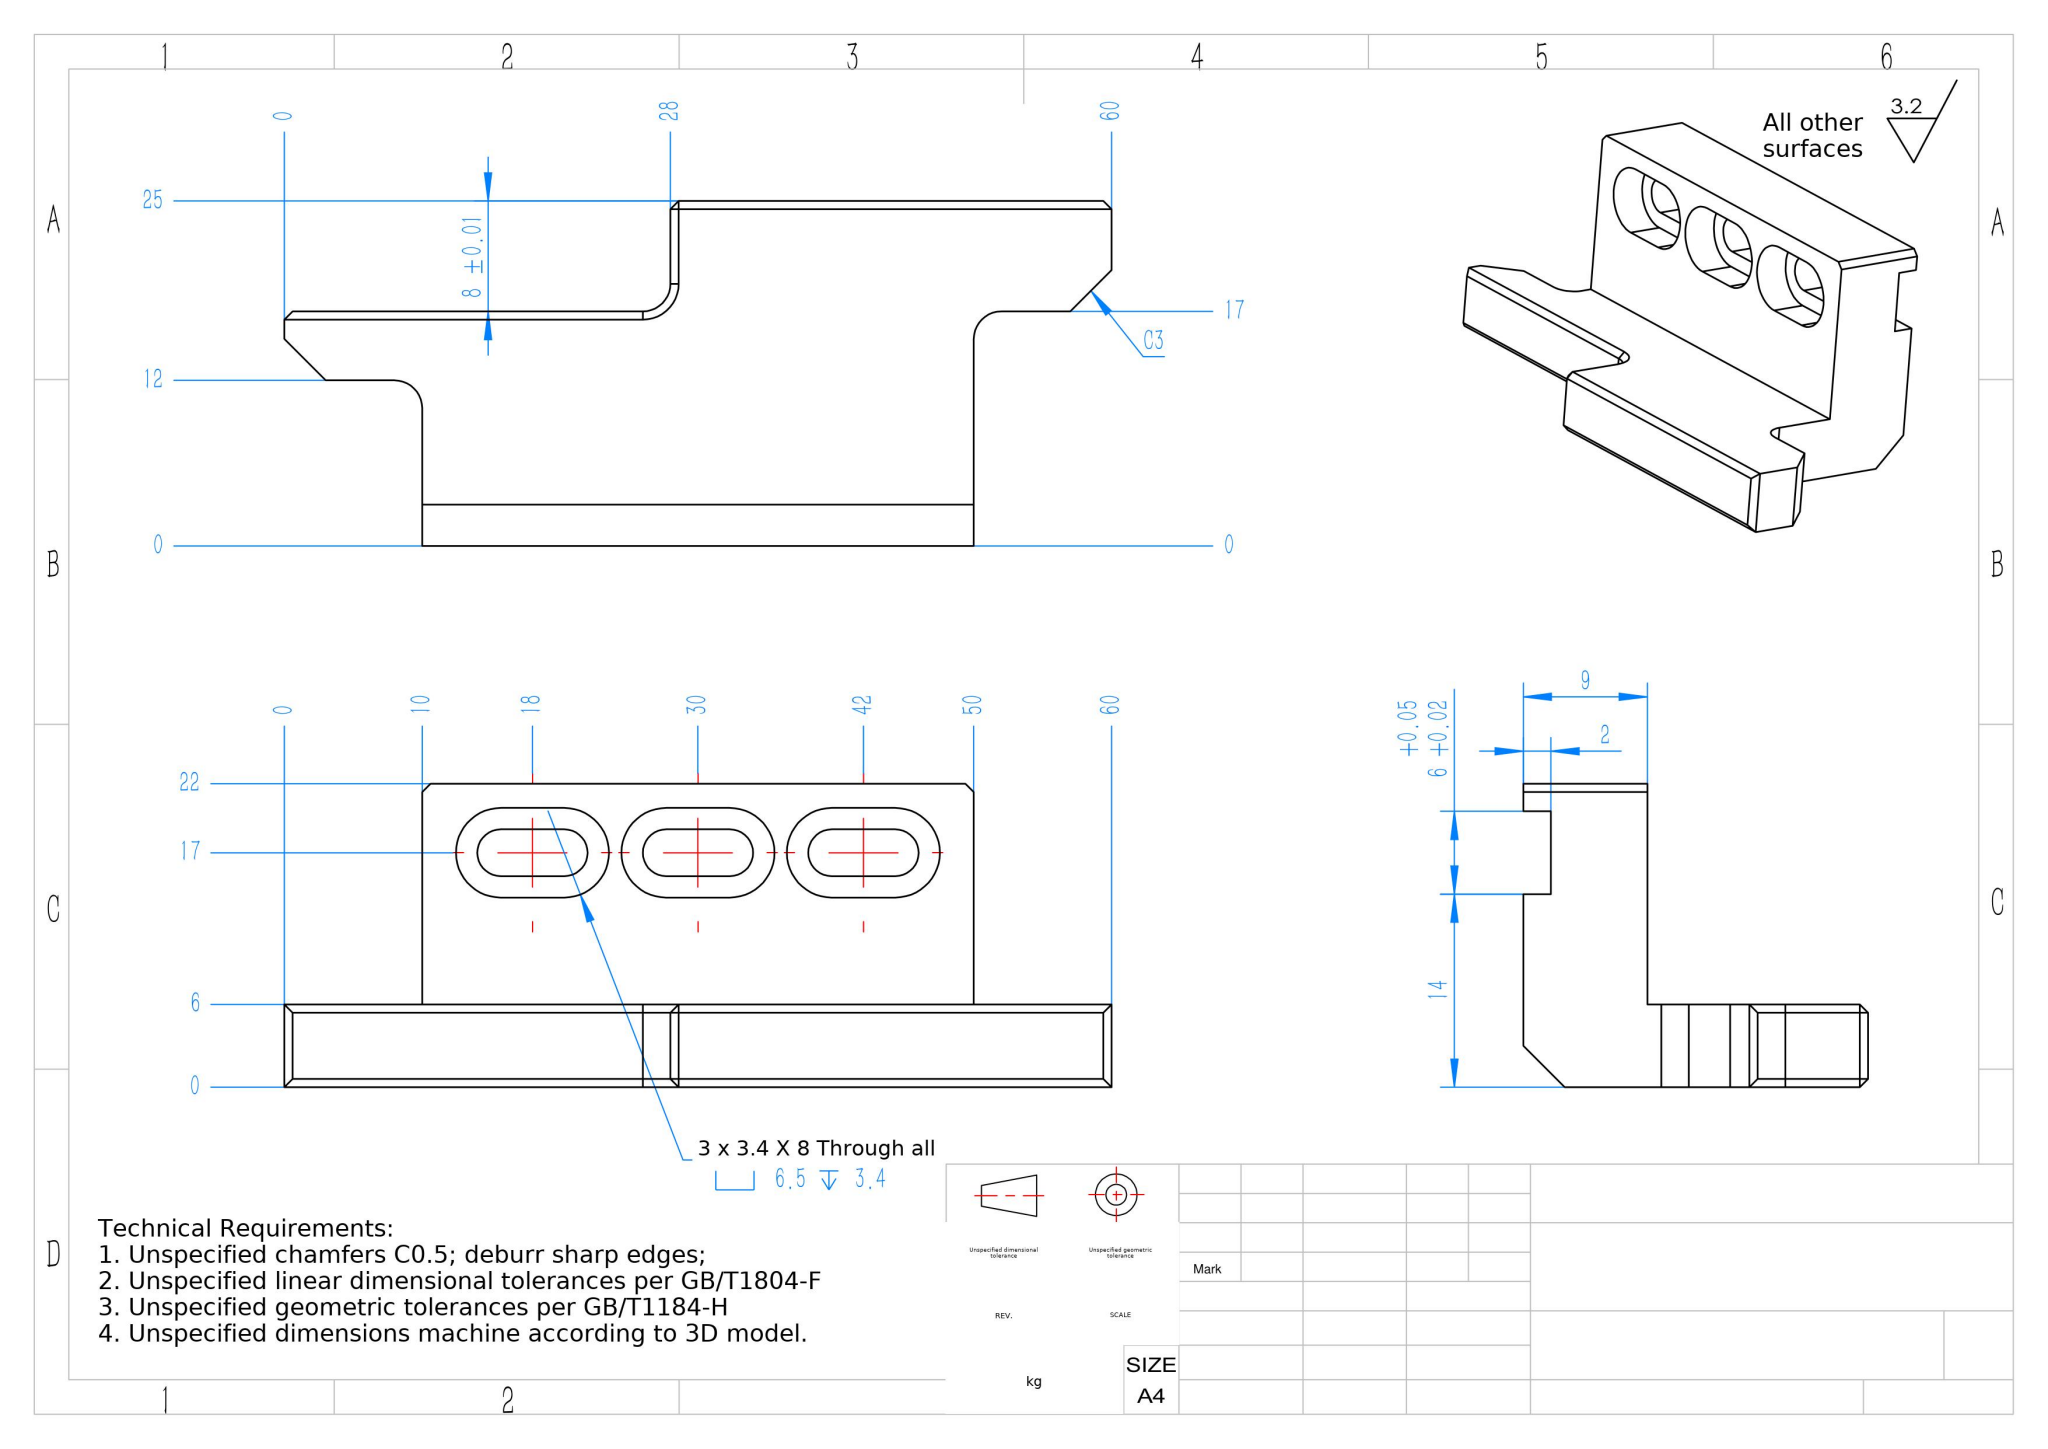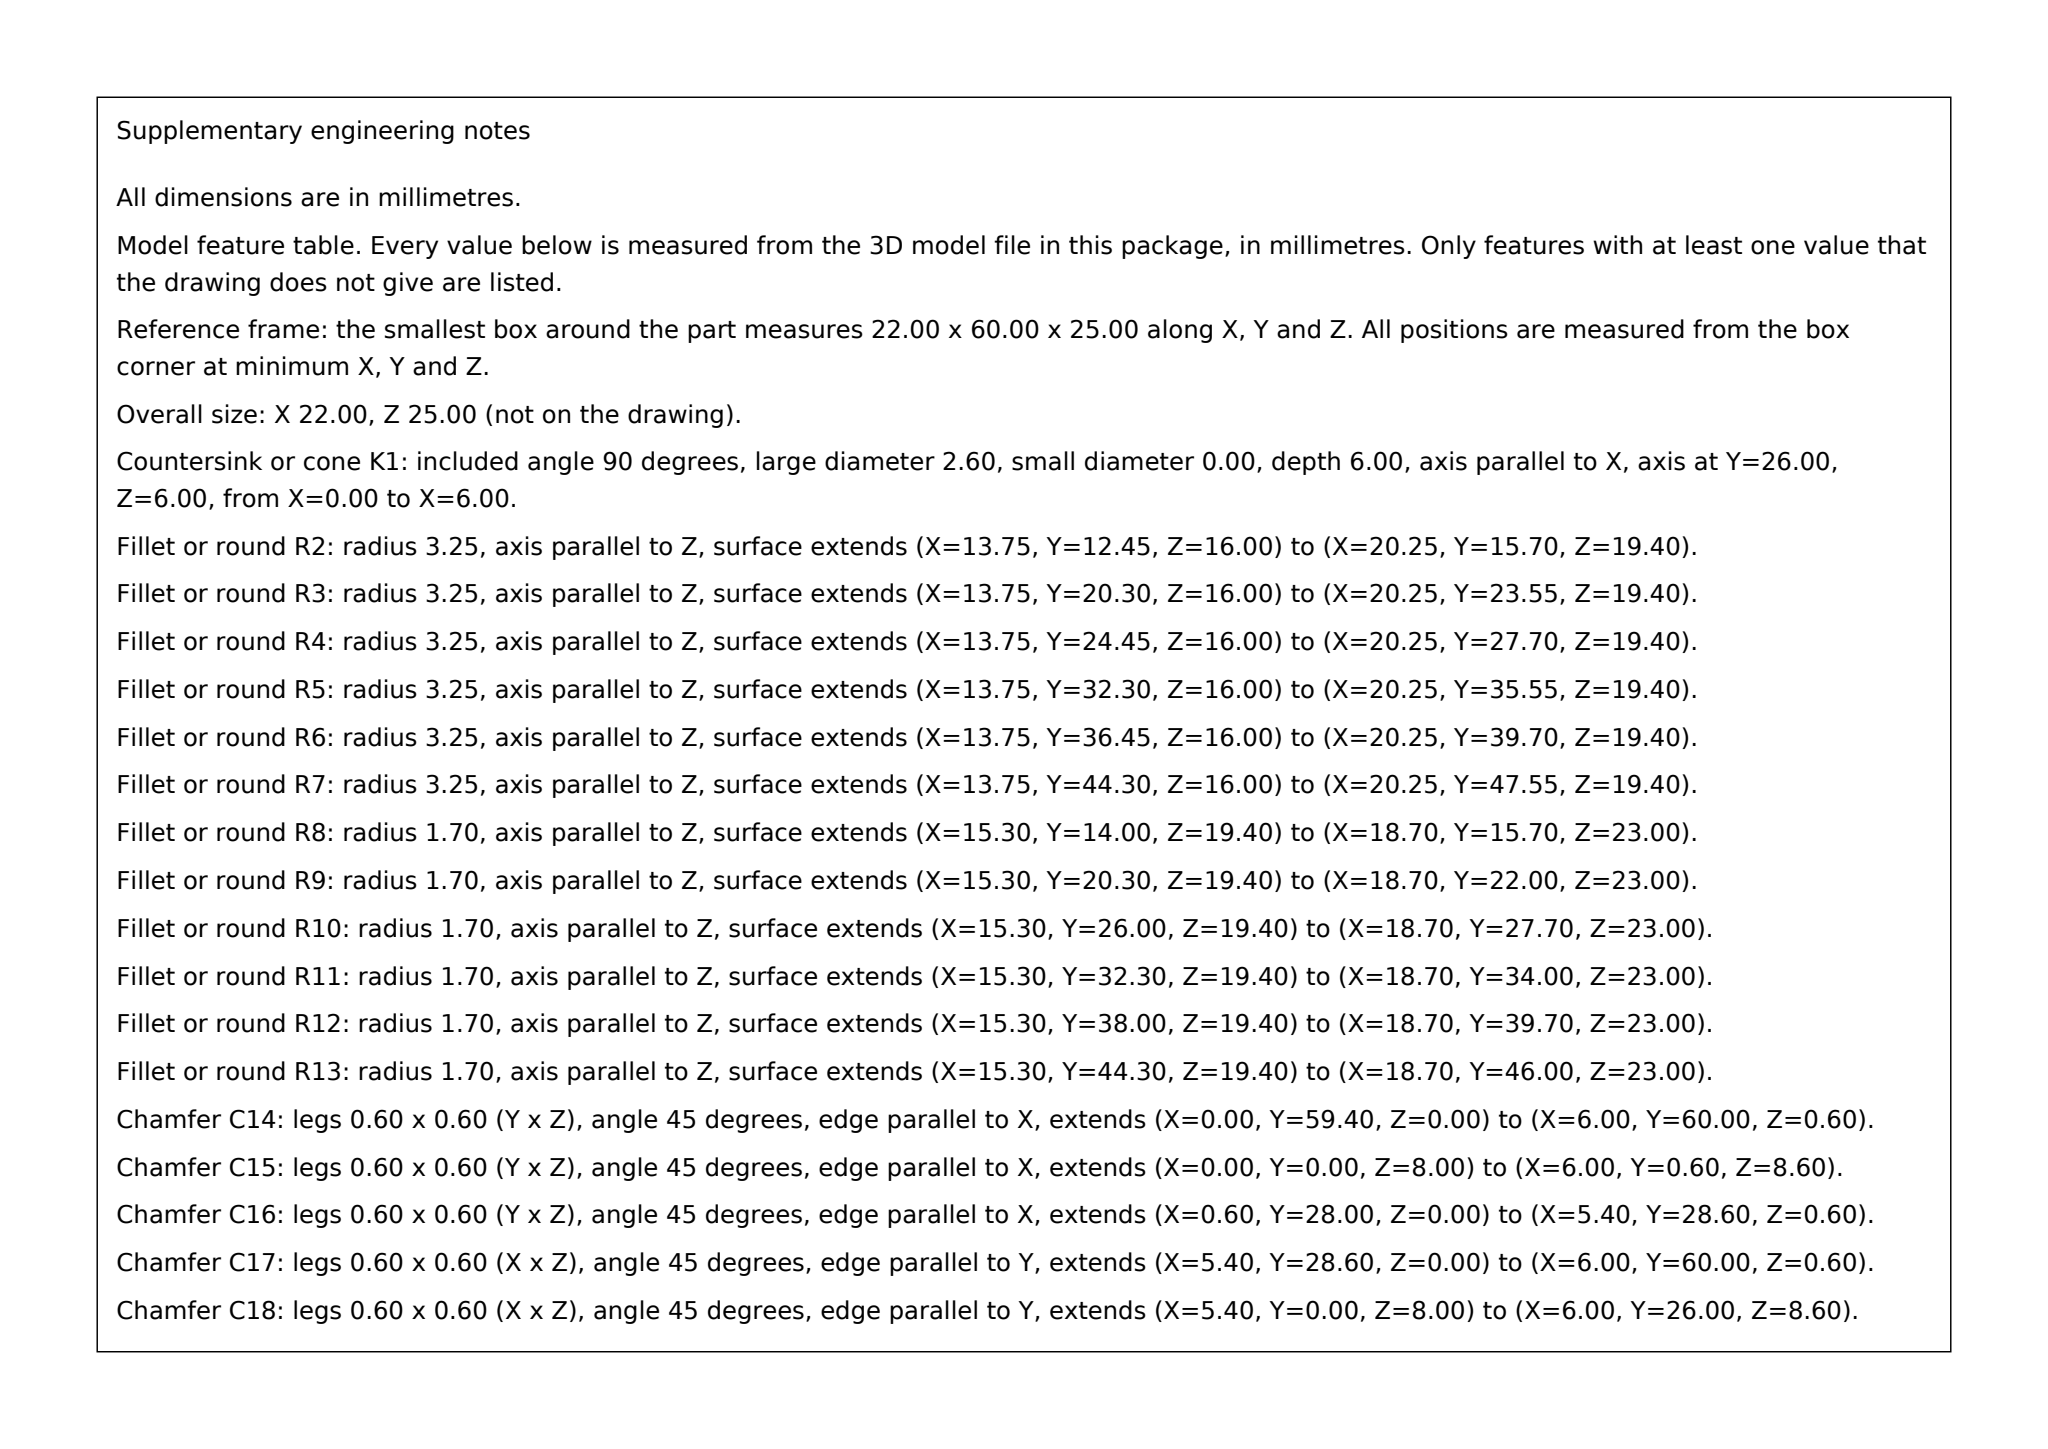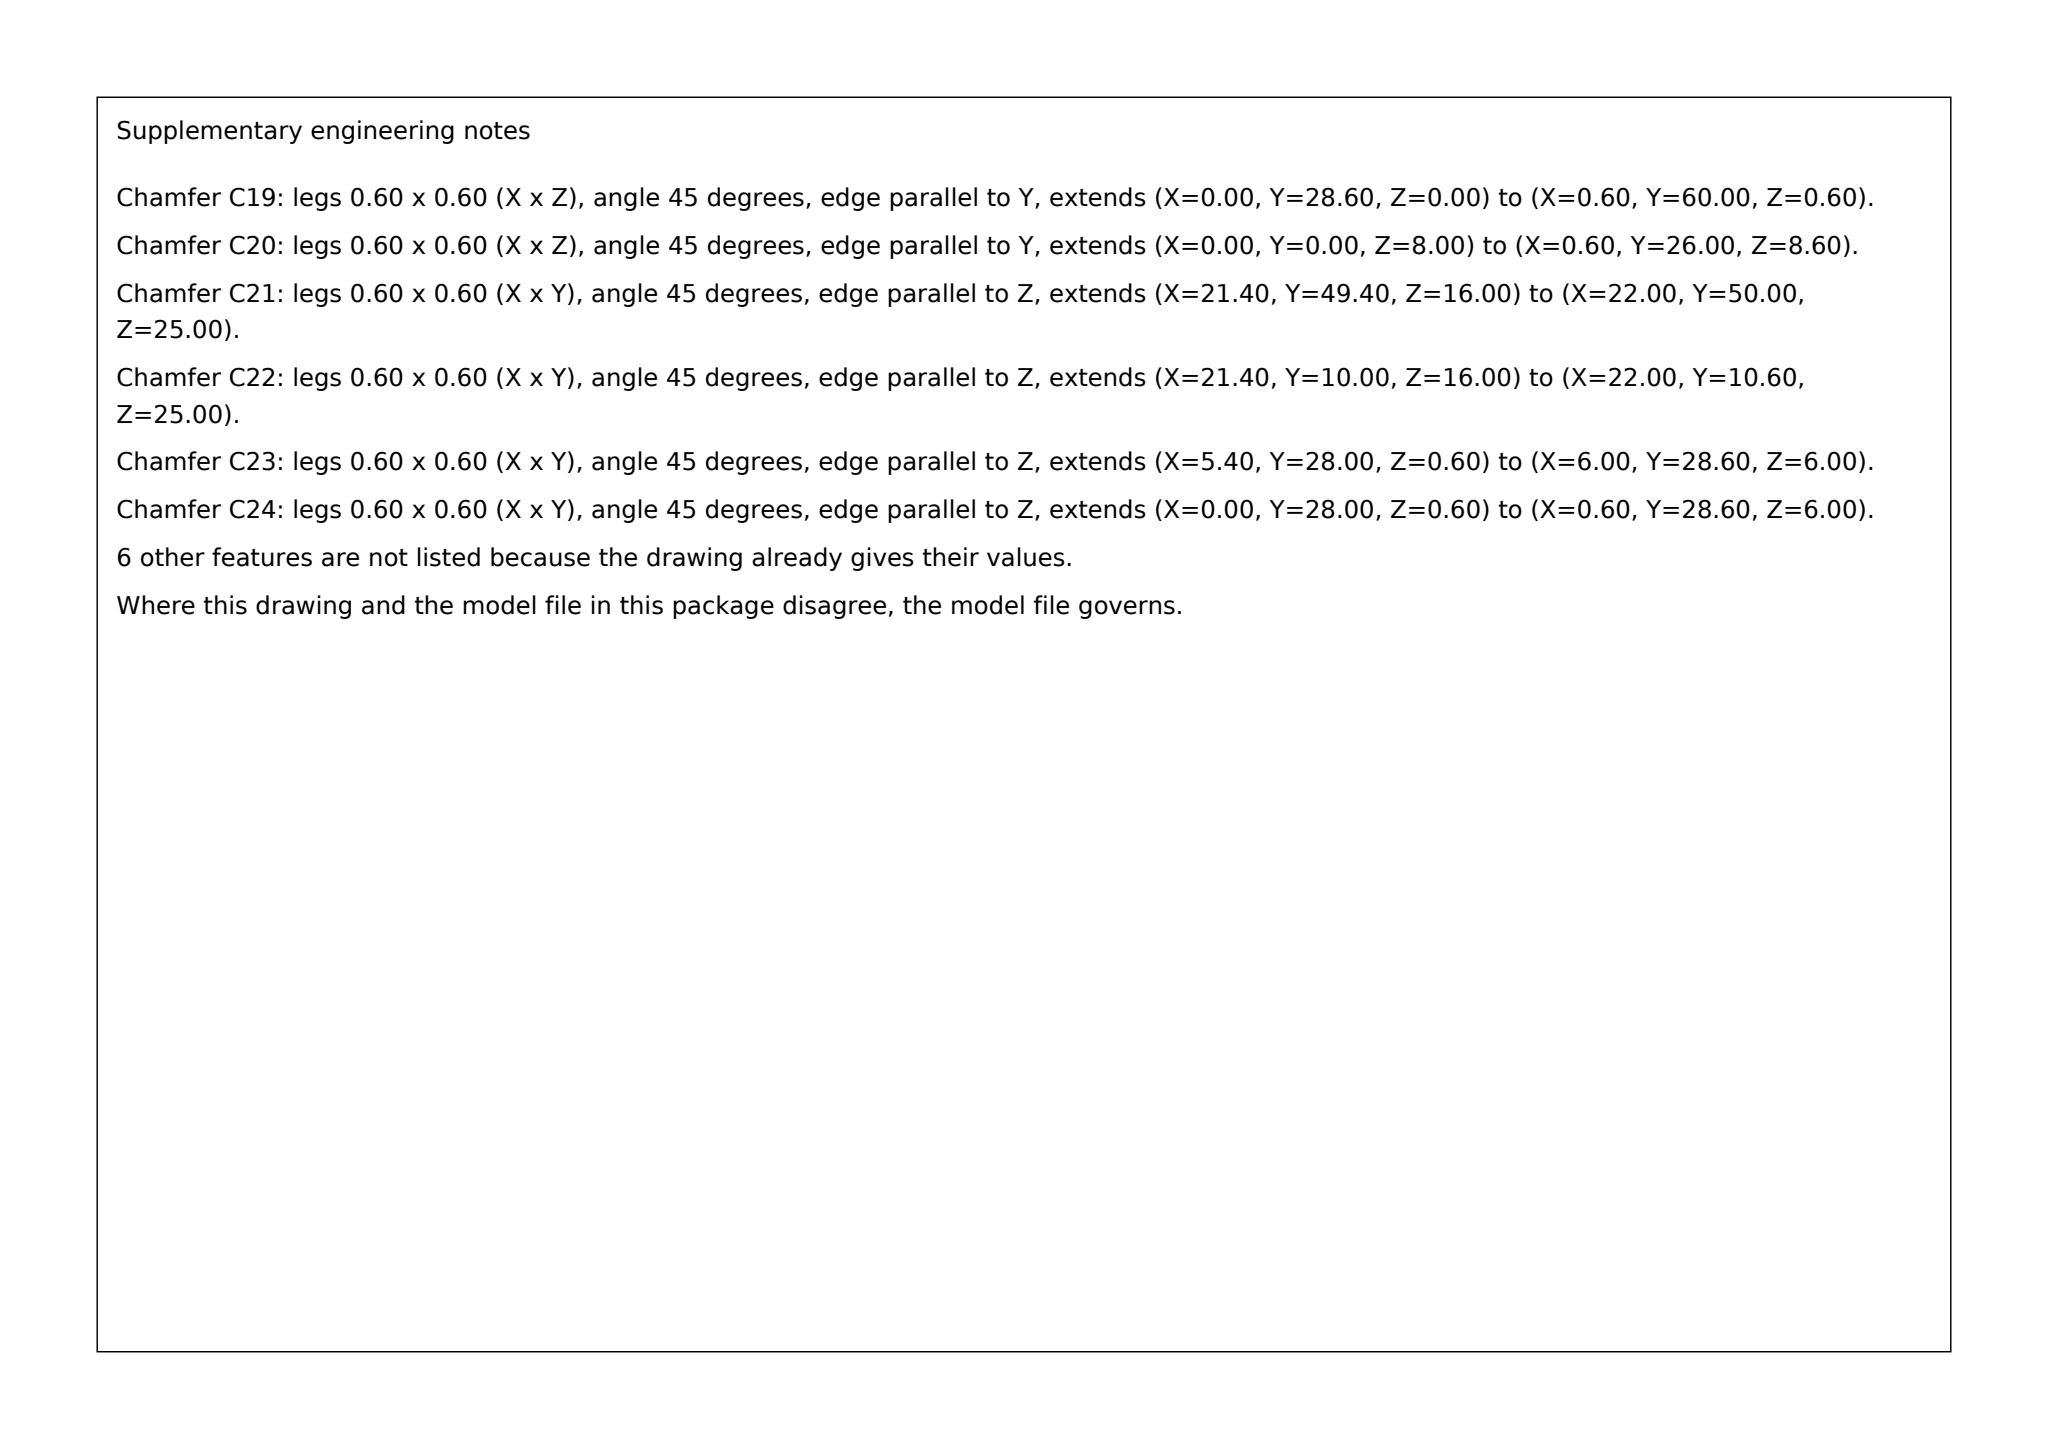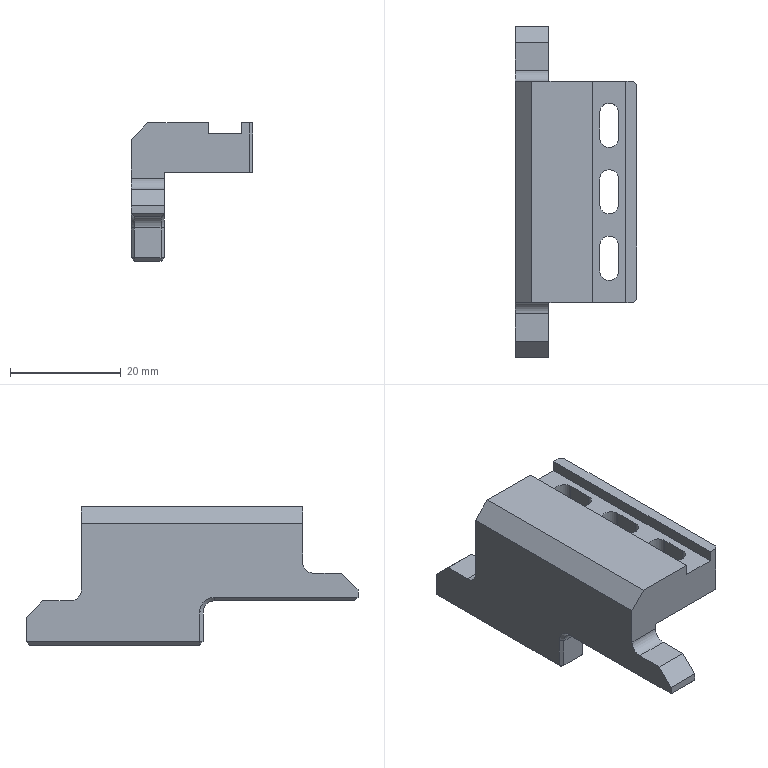Part | SolidWorks | 1 solid | 66 faces | box 22 x 60 x 25 mm | volume 10037 mm3 | plane 49 | cylinder 15 | cone 2 | commonest cylinder face diameters 3.4 x6 6.5 x6 4 x3